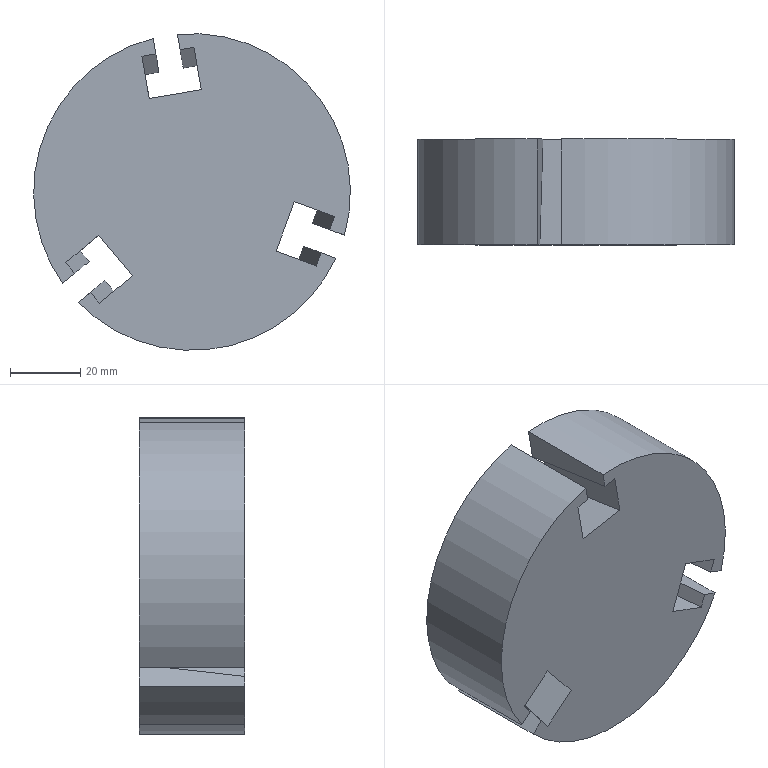Component | SolidWorks | K51-2_K51-3-1 | 1 solid | 27 faces | box 90 x 30 x 90 mm | volume 169880 mm3 | plane 23 | cylinder 4 | commonest cylinder face diameters 90 x4
STEP:
#1=COLOUR_RGB('',0.7922,0.8196,0.9333);
#2=FILL_AREA_STYLE_COLOUR('',#1);
#3=FILL_AREA_STYLE('',(#2));
#4=SURFACE_STYLE_FILL_AREA(#3);
#5=SURFACE_SIDE_STYLE('',(#4));
#6=SURFACE_STYLE_USAGE(.BOTH.,#5);
#7=PRESENTATION_STYLE_ASSIGNMENT((#6));
#8=CARTESIAN_POINT('',(-10.063,38.924,1.881));
#9=VERTEX_POINT('',#8);
#10=CARTESIAN_POINT('',(-10.719,38.924,2.308));
#11=VERTEX_POINT('',#10);
#12=CARTESIAN_POINT('',(-9.449,38.924,3.543));
#13=DIRECTION('',(0.,1.,0.));
#14=DIRECTION('',(0.3464,0.,0.9381));
#15=AXIS2_PLACEMENT_3D('',#12,#13,#14);
#16=CIRCLE('',#15,1.772);
#17=EDGE_CURVE('',#9,#11,#16,.T.);
#18=ORIENTED_EDGE('',*,*,#17,.F.);
#19=CARTESIAN_POINT('',(-10.063,37.743,1.881));
#20=VERTEX_POINT('',#19);
#21=CARTESIAN_POINT('',(-10.063,38.924,1.881));
#22=DIRECTION('',(0.,-1.,0.));
#23=VECTOR('',#22,39.37);
#24=LINE('',#21,#23);
#25=EDGE_CURVE('',#9,#20,#24,.T.);
#26=ORIENTED_EDGE('',*,*,#25,.T.);
#27=CARTESIAN_POINT('',(-10.719,37.743,2.308));
#28=VERTEX_POINT('',#27);
#29=CARTESIAN_POINT('',(-9.449,37.743,3.543));
#30=DIRECTION('',(0.,1.,0.));
#31=DIRECTION('',(0.3464,0.,0.9381));
#32=AXIS2_PLACEMENT_3D('',#29,#30,#31);
#33=CIRCLE('',#32,1.772);
#34=EDGE_CURVE('',#20,#28,#33,.T.);
#35=ORIENTED_EDGE('',*,*,#34,.T.);
#36=CARTESIAN_POINT('',(-10.719,38.924,2.308));
#37=DIRECTION('',(0.,1.,0.));
#38=VECTOR('',#37,39.37);
#39=LINE('',#36,#38);
#40=EDGE_CURVE('',#28,#11,#39,.T.);
#41=ORIENTED_EDGE('',*,*,#40,.T.);
#42=EDGE_LOOP('',(#18,#26,#35,#41));
#43=FACE_OUTER_BOUND('',#42,.T.);
#44=CARTESIAN_POINT('',(-9.449,38.924,3.543));
#45=DIRECTION('',(0.,-1.,0.));
#46=DIRECTION('',(-0.3464,0.,-0.9381));
#47=AXIS2_PLACEMENT_3D('',#44,#45,#46);
#48=CYLINDRICAL_SURFACE('',#47,1.772);
#49=ADVANCED_FACE('',(#43),#48,.T.);
#50=CARTESIAN_POINT('',(-10.895,38.924,2.52));
#51=VERTEX_POINT('',#50);
#52=CARTESIAN_POINT('',(-9.883,38.924,5.261));
#53=VERTEX_POINT('',#52);
#54=CARTESIAN_POINT('',(-9.449,38.924,3.543));
#55=DIRECTION('',(0.,1.,0.));
#56=DIRECTION('',(0.3464,0.,0.9381));
#57=AXIS2_PLACEMENT_3D('',#54,#55,#56);
#58=CIRCLE('',#57,1.772);
#59=EDGE_CURVE('',#51,#53,#58,.T.);
#60=ORIENTED_EDGE('',*,*,#59,.F.);
#61=CARTESIAN_POINT('',(-10.895,37.743,2.52));
#62=VERTEX_POINT('',#61);
#63=CARTESIAN_POINT('',(-10.895,38.924,2.52));
#64=DIRECTION('',(0.,-1.,0.));
#65=VECTOR('',#64,39.37);
#66=LINE('',#63,#65);
#67=EDGE_CURVE('',#51,#62,#66,.T.);
#68=ORIENTED_EDGE('',*,*,#67,.T.);
#69=CARTESIAN_POINT('',(-9.883,37.743,5.261));
#70=VERTEX_POINT('',#69);
#71=CARTESIAN_POINT('',(-9.449,37.743,3.543));
#72=DIRECTION('',(0.,1.,0.));
#73=DIRECTION('',(0.3464,0.,0.9381));
#74=AXIS2_PLACEMENT_3D('',#71,#72,#73);
#75=CIRCLE('',#74,1.772);
#76=EDGE_CURVE('',#62,#70,#75,.T.);
#77=ORIENTED_EDGE('',*,*,#76,.T.);
#78=CARTESIAN_POINT('',(-9.883,38.924,5.261));
#79=DIRECTION('',(0.,1.,0.));
#80=VECTOR('',#79,39.37);
#81=LINE('',#78,#80);
#82=EDGE_CURVE('',#70,#53,#81,.T.);
#83=ORIENTED_EDGE('',*,*,#82,.T.);
#84=EDGE_LOOP('',(#60,#68,#77,#83));
#85=FACE_OUTER_BOUND('',#84,.T.);
#86=CARTESIAN_POINT('',(-9.449,38.924,3.543));
#87=DIRECTION('',(0.,-1.,0.));
#88=DIRECTION('',(-0.3464,0.,-0.9381));
#89=AXIS2_PLACEMENT_3D('',#86,#87,#88);
#90=CYLINDRICAL_SURFACE('',#89,1.772);
#91=ADVANCED_FACE('',(#85),#90,.T.);
#92=CARTESIAN_POINT('',(-9.612,38.924,5.307));
#93=VERTEX_POINT('',#92);
#94=CARTESIAN_POINT('',(-7.744,38.924,3.061));
#95=VERTEX_POINT('',#94);
#96=CARTESIAN_POINT('',(-9.449,38.924,3.543));
#97=DIRECTION('',(0.,1.,0.));
#98=DIRECTION('',(0.3464,0.,0.9381));
#99=AXIS2_PLACEMENT_3D('',#96,#97,#98);
#100=CIRCLE('',#99,1.772);
#101=EDGE_CURVE('',#93,#95,#100,.T.);
#102=ORIENTED_EDGE('',*,*,#101,.F.);
#103=CARTESIAN_POINT('',(-9.612,37.743,5.307));
#104=VERTEX_POINT('',#103);
#105=CARTESIAN_POINT('',(-9.612,38.924,5.307));
#106=DIRECTION('',(0.,-1.,0.));
#107=VECTOR('',#106,39.37);
#108=LINE('',#105,#107);
#109=EDGE_CURVE('',#93,#104,#108,.T.);
#110=ORIENTED_EDGE('',*,*,#109,.T.);
#111=CARTESIAN_POINT('',(-7.744,37.743,3.061));
#112=VERTEX_POINT('',#111);
#113=CARTESIAN_POINT('',(-9.449,37.743,3.543));
#114=DIRECTION('',(0.,1.,0.));
#115=DIRECTION('',(0.3464,0.,0.9381));
#116=AXIS2_PLACEMENT_3D('',#113,#114,#115);
#117=CIRCLE('',#116,1.772);
#118=EDGE_CURVE('',#104,#112,#117,.T.);
#119=ORIENTED_EDGE('',*,*,#118,.T.);
#120=CARTESIAN_POINT('',(-7.744,38.924,3.061));
#121=DIRECTION('',(0.,1.,0.));
#122=VECTOR('',#121,39.37);
#123=LINE('',#120,#122);
#124=EDGE_CURVE('',#112,#95,#123,.T.);
#125=ORIENTED_EDGE('',*,*,#124,.T.);
#126=EDGE_LOOP('',(#102,#110,#119,#125));
#127=FACE_OUTER_BOUND('',#126,.T.);
#128=CARTESIAN_POINT('',(-9.449,38.924,3.543));
#129=DIRECTION('',(0.,-1.,0.));
#130=DIRECTION('',(-0.3464,0.,-0.9381));
#131=AXIS2_PLACEMENT_3D('',#128,#129,#130);
#132=CYLINDRICAL_SURFACE('',#131,1.772);
#133=ADVANCED_FACE('',(#127),#132,.T.);
#134=ORIENTED_EDGE('',*,*,#25,.F.);
#135=CARTESIAN_POINT('',(-7.84,38.924,2.802));
#136=VERTEX_POINT('',#135);
#137=CARTESIAN_POINT('',(-9.449,38.924,3.543));
#138=DIRECTION('',(0.,1.,0.));
#139=DIRECTION('',(0.3464,0.,0.9381));
#140=AXIS2_PLACEMENT_3D('',#137,#138,#139);
#141=CIRCLE('',#140,1.772);
#142=EDGE_CURVE('',#136,#9,#141,.T.);
#143=ORIENTED_EDGE('',*,*,#142,.F.);
#144=CARTESIAN_POINT('',(-7.84,37.743,2.802));
#145=VERTEX_POINT('',#144);
#146=CARTESIAN_POINT('',(-7.84,38.924,2.802));
#147=DIRECTION('',(0.,-1.,0.));
#148=VECTOR('',#147,39.37);
#149=LINE('',#146,#148);
#150=EDGE_CURVE('',#136,#145,#149,.T.);
#151=ORIENTED_EDGE('',*,*,#150,.T.);
#152=CARTESIAN_POINT('',(-9.449,37.743,3.543));
#153=DIRECTION('',(0.,1.,0.));
#154=DIRECTION('',(0.3464,0.,0.9381));
#155=AXIS2_PLACEMENT_3D('',#152,#153,#154);
#156=CIRCLE('',#155,1.772);
#157=EDGE_CURVE('',#145,#20,#156,.T.);
#158=ORIENTED_EDGE('',*,*,#157,.T.);
#159=EDGE_LOOP('',(#134,#143,#151,#158));
#160=FACE_OUTER_BOUND('',#159,.T.);
#161=CARTESIAN_POINT('',(-9.449,38.924,3.543));
#162=DIRECTION('',(0.,-1.,0.));
#163=DIRECTION('',(-0.3464,0.,-0.9381));
#164=AXIS2_PLACEMENT_3D('',#161,#162,#163);
#165=CYLINDRICAL_SURFACE('',#164,1.772);
#166=ADVANCED_FACE('',(#160),#165,.T.);
#167=CARTESIAN_POINT('',(-10.601,38.924,2.765));
#168=VERTEX_POINT('',#167);
#169=CARTESIAN_POINT('',(-9.537,38.924,3.649));
#170=DIRECTION('',(0.769,0.,0.6392));
#171=VECTOR('',#170,39.37);
#172=LINE('',#169,#171);
#173=EDGE_CURVE('',#51,#168,#172,.T.);
#174=ORIENTED_EDGE('',*,*,#173,.F.);
#175=ORIENTED_EDGE('',*,*,#59,.T.);
#176=CARTESIAN_POINT('',(-9.818,38.924,4.883));
#177=VERTEX_POINT('',#176);
#178=CARTESIAN_POINT('',(-9.585,38.924,3.52));
#179=DIRECTION('',(-0.169,0.,0.9856));
#180=VECTOR('',#179,39.37);
#181=LINE('',#178,#180);
#182=EDGE_CURVE('',#177,#53,#181,.T.);
#183=ORIENTED_EDGE('',*,*,#182,.F.);
#184=CARTESIAN_POINT('',(-9.974,38.924,4.857));
#185=VERTEX_POINT('',#184);
#186=CARTESIAN_POINT('',(-9.683,38.924,4.907));
#187=DIRECTION('',(0.9856,0.,0.169));
#188=VECTOR('',#187,39.37);
#189=LINE('',#186,#188);
#190=EDGE_CURVE('',#185,#177,#189,.T.);
#191=ORIENTED_EDGE('',*,*,#190,.F.);
#192=CARTESIAN_POINT('',(-9.893,38.924,4.384));
#193=VERTEX_POINT('',#192);
#194=CARTESIAN_POINT('',(-9.74,38.924,3.493));
#195=DIRECTION('',(-0.169,0.,0.9856));
#196=VECTOR('',#195,39.37);
#197=LINE('',#194,#196);
#198=EDGE_CURVE('',#193,#185,#197,.T.);
#199=ORIENTED_EDGE('',*,*,#198,.F.);
#200=CARTESIAN_POINT('',(-9.31,38.924,4.484));
#201=VERTEX_POINT('',#200);
#202=CARTESIAN_POINT('',(-9.602,38.924,4.434));
#203=DIRECTION('',(-0.9856,0.,-0.169));
#204=VECTOR('',#203,39.37);
#205=LINE('',#202,#204);
#206=EDGE_CURVE('',#201,#193,#205,.T.);
#207=ORIENTED_EDGE('',*,*,#206,.F.);
#208=CARTESIAN_POINT('',(-9.392,38.924,4.956));
#209=VERTEX_POINT('',#208);
#210=CARTESIAN_POINT('',(-9.158,38.924,3.593));
#211=DIRECTION('',(0.169,0.,-0.9856));
#212=VECTOR('',#211,39.37);
#213=LINE('',#210,#212);
#214=EDGE_CURVE('',#209,#201,#213,.T.);
#215=ORIENTED_EDGE('',*,*,#214,.F.);
#216=CARTESIAN_POINT('',(-9.547,38.924,4.93));
#217=VERTEX_POINT('',#216);
#218=CARTESIAN_POINT('',(-9.683,38.924,4.907));
#219=DIRECTION('',(0.9856,0.,0.169));
#220=VECTOR('',#219,39.37);
#221=LINE('',#218,#220);
#222=EDGE_CURVE('',#217,#209,#221,.T.);
#223=ORIENTED_EDGE('',*,*,#222,.F.);
#224=CARTESIAN_POINT('',(-9.313,38.924,3.567));
#225=DIRECTION('',(0.169,0.,-0.9856));
#226=VECTOR('',#225,39.37);
#227=LINE('',#224,#226);
#228=EDGE_CURVE('',#93,#217,#227,.T.);
#229=ORIENTED_EDGE('',*,*,#228,.F.);
#230=ORIENTED_EDGE('',*,*,#101,.T.);
#231=CARTESIAN_POINT('',(-8.104,38.924,3.193));
#232=VERTEX_POINT('',#231);
#233=CARTESIAN_POINT('',(-9.401,38.924,3.673));
#234=DIRECTION('',(0.9381,0.,-0.3464));
#235=VECTOR('',#234,39.37);
#236=LINE('',#233,#235);
#237=EDGE_CURVE('',#232,#95,#236,.T.);
#238=ORIENTED_EDGE('',*,*,#237,.F.);
#239=CARTESIAN_POINT('',(-8.049,38.924,3.341));
#240=VERTEX_POINT('',#239);
#241=CARTESIAN_POINT('',(-8.151,38.924,3.064));
#242=DIRECTION('',(-0.3464,0.,-0.9381));
#243=VECTOR('',#242,39.37);
#244=LINE('',#241,#243);
#245=EDGE_CURVE('',#240,#232,#244,.T.);
#246=ORIENTED_EDGE('',*,*,#245,.F.);
#247=CARTESIAN_POINT('',(-8.499,38.924,3.507));
#248=VERTEX_POINT('',#247);
#249=CARTESIAN_POINT('',(-9.347,38.924,3.82));
#250=DIRECTION('',(0.9381,0.,-0.3464));
#251=VECTOR('',#250,39.37);
#252=LINE('',#249,#251);
#253=EDGE_CURVE('',#248,#240,#252,.T.);
#254=ORIENTED_EDGE('',*,*,#253,.F.);
#255=CARTESIAN_POINT('',(-8.704,38.924,2.953));
#256=VERTEX_POINT('',#255);
#257=CARTESIAN_POINT('',(-8.601,38.924,3.23));
#258=DIRECTION('',(0.3464,0.,0.9381));
#259=VECTOR('',#258,39.37);
#260=LINE('',#257,#259);
#261=EDGE_CURVE('',#256,#248,#260,.T.);
#262=ORIENTED_EDGE('',*,*,#261,.F.);
#263=CARTESIAN_POINT('',(-8.254,38.924,2.787));
#264=VERTEX_POINT('',#263);
#265=CARTESIAN_POINT('',(-9.551,38.924,3.266));
#266=DIRECTION('',(-0.9381,0.,0.3464));
#267=VECTOR('',#266,39.37);
#268=LINE('',#265,#267);
#269=EDGE_CURVE('',#264,#256,#268,.T.);
#270=ORIENTED_EDGE('',*,*,#269,.F.);
#271=CARTESIAN_POINT('',(-8.199,38.924,2.935));
#272=VERTEX_POINT('',#271);
#273=CARTESIAN_POINT('',(-8.151,38.924,3.064));
#274=DIRECTION('',(-0.3464,0.,-0.9381));
#275=VECTOR('',#274,39.37);
#276=LINE('',#273,#275);
#277=EDGE_CURVE('',#272,#264,#276,.T.);
#278=ORIENTED_EDGE('',*,*,#277,.F.);
#279=CARTESIAN_POINT('',(-9.497,38.924,3.414));
#280=DIRECTION('',(-0.9381,0.,0.3464));
#281=VECTOR('',#280,39.37);
#282=LINE('',#279,#281);
#283=EDGE_CURVE('',#136,#272,#282,.T.);
#284=ORIENTED_EDGE('',*,*,#283,.F.);
#285=ORIENTED_EDGE('',*,*,#142,.T.);
#286=ORIENTED_EDGE('',*,*,#17,.T.);
#287=CARTESIAN_POINT('',(-10.424,38.924,2.553));
#288=VERTEX_POINT('',#287);
#289=CARTESIAN_POINT('',(-9.361,38.924,3.437));
#290=DIRECTION('',(-0.769,0.,-0.6392));
#291=VECTOR('',#290,39.37);
#292=LINE('',#289,#291);
#293=EDGE_CURVE('',#288,#11,#292,.T.);
#294=ORIENTED_EDGE('',*,*,#293,.F.);
#295=CARTESIAN_POINT('',(-10.324,38.924,2.432));
#296=VERTEX_POINT('',#295);
#297=CARTESIAN_POINT('',(-10.513,38.924,2.659));
#298=DIRECTION('',(-0.6392,0.,0.769));
#299=VECTOR('',#298,39.37);
#300=LINE('',#297,#299);
#301=EDGE_CURVE('',#296,#288,#300,.T.);
#302=ORIENTED_EDGE('',*,*,#301,.F.);
#303=CARTESIAN_POINT('',(-9.955,38.924,2.739));
#304=VERTEX_POINT('',#303);
#305=CARTESIAN_POINT('',(-9.26,38.924,3.316));
#306=DIRECTION('',(-0.769,0.,-0.6392));
#307=VECTOR('',#306,39.37);
#308=LINE('',#305,#307);
#309=EDGE_CURVE('',#304,#296,#308,.T.);
#310=ORIENTED_EDGE('',*,*,#309,.F.);
#311=CARTESIAN_POINT('',(-10.332,38.924,3.193));
#312=VERTEX_POINT('',#311);
#313=CARTESIAN_POINT('',(-10.144,38.924,2.966));
#314=DIRECTION('',(0.6392,0.,-0.769));
#315=VECTOR('',#314,39.37);
#316=LINE('',#313,#315);
#317=EDGE_CURVE('',#312,#304,#316,.T.);
#318=ORIENTED_EDGE('',*,*,#317,.F.);
#319=CARTESIAN_POINT('',(-10.701,38.924,2.886));
#320=VERTEX_POINT('',#319);
#321=CARTESIAN_POINT('',(-9.638,38.924,3.77));
#322=DIRECTION('',(0.769,0.,0.6392));
#323=VECTOR('',#322,39.37);
#324=LINE('',#321,#323);
#325=EDGE_CURVE('',#320,#312,#324,.T.);
#326=ORIENTED_EDGE('',*,*,#325,.F.);
#327=CARTESIAN_POINT('',(-10.513,38.924,2.659));
#328=DIRECTION('',(-0.6392,0.,0.769));
#329=VECTOR('',#328,39.37);
#330=LINE('',#327,#329);
#331=EDGE_CURVE('',#168,#320,#330,.T.);
#332=ORIENTED_EDGE('',*,*,#331,.F.);
#333=EDGE_LOOP('',(#174,#175,#183,#191,#199,#207,#215,#223,#229,#230,#238,#246,#254,#262,#270,#278,#284,#285,#286,#294,#302,#310,#318,#326,#332));
#334=FACE_OUTER_BOUND('',#333,.T.);
#335=CARTESIAN_POINT('',(-9.449,38.924,3.543));
#336=DIRECTION('',(0.,1.,0.));
#337=DIRECTION('',(0.3464,0.,0.9381));
#338=AXIS2_PLACEMENT_3D('',#335,#336,#337);
#339=PLANE('',#338);
#340=ADVANCED_FACE('',(#334),#339,.T.);
#341=ORIENTED_EDGE('',*,*,#76,.F.);
#342=CARTESIAN_POINT('',(-10.761,37.743,2.632));
#343=VERTEX_POINT('',#342);
#344=CARTESIAN_POINT('',(-9.537,37.743,3.649));
#345=DIRECTION('',(0.769,0.,0.6392));
#346=VECTOR('',#345,39.37);
#347=LINE('',#344,#346);
#348=EDGE_CURVE('',#62,#343,#347,.T.);
#349=ORIENTED_EDGE('',*,*,#348,.T.);
#350=CARTESIAN_POINT('',(-10.861,37.743,2.753));
#351=VERTEX_POINT('',#350);
#352=CARTESIAN_POINT('',(-10.673,37.743,2.526));
#353=DIRECTION('',(-0.6392,0.,0.769));
#354=VECTOR('',#353,39.37);
#355=LINE('',#352,#354);
#356=EDGE_CURVE('',#343,#351,#355,.T.);
#357=ORIENTED_EDGE('',*,*,#356,.T.);
#358=CARTESIAN_POINT('',(-10.492,37.743,3.06));
#359=VERTEX_POINT('',#358);
#360=CARTESIAN_POINT('',(-9.638,37.743,3.77));
#361=DIRECTION('',(0.769,0.,0.6392));
#362=VECTOR('',#361,39.37);
#363=LINE('',#360,#362);
#364=EDGE_CURVE('',#351,#359,#363,.T.);
#365=ORIENTED_EDGE('',*,*,#364,.T.);
#366=CARTESIAN_POINT('',(-10.115,37.743,2.606));
#367=VERTEX_POINT('',#366);
#368=CARTESIAN_POINT('',(-10.304,37.743,2.833));
#369=DIRECTION('',(0.6392,0.,-0.769));
#370=VECTOR('',#369,39.37);
#371=LINE('',#368,#370);
#372=EDGE_CURVE('',#359,#367,#371,.T.);
#373=ORIENTED_EDGE('',*,*,#372,.T.);
#374=CARTESIAN_POINT('',(-10.484,37.743,2.299));
#375=VERTEX_POINT('',#374);
#376=CARTESIAN_POINT('',(-9.26,37.743,3.316));
#377=DIRECTION('',(-0.769,0.,-0.6392));
#378=VECTOR('',#377,39.37);
#379=LINE('',#376,#378);
#380=EDGE_CURVE('',#367,#375,#379,.T.);
#381=ORIENTED_EDGE('',*,*,#380,.T.);
#382=CARTESIAN_POINT('',(-10.585,37.743,2.42));
#383=VERTEX_POINT('',#382);
#384=CARTESIAN_POINT('',(-10.673,37.743,2.526));
#385=DIRECTION('',(-0.6392,0.,0.769));
#386=VECTOR('',#385,39.37);
#387=LINE('',#384,#386);
#388=EDGE_CURVE('',#375,#383,#387,.T.);
#389=ORIENTED_EDGE('',*,*,#388,.T.);
#390=CARTESIAN_POINT('',(-9.361,37.743,3.437));
#391=DIRECTION('',(-0.769,0.,-0.6392));
#392=VECTOR('',#391,39.37);
#393=LINE('',#390,#392);
#394=EDGE_CURVE('',#383,#28,#393,.T.);
#395=ORIENTED_EDGE('',*,*,#394,.T.);
#396=ORIENTED_EDGE('',*,*,#34,.F.);
#397=ORIENTED_EDGE('',*,*,#157,.F.);
#398=CARTESIAN_POINT('',(-8.004,37.743,2.863));
#399=VERTEX_POINT('',#398);
#400=CARTESIAN_POINT('',(-9.497,37.743,3.414));
#401=DIRECTION('',(-0.9381,0.,0.3464));
#402=VECTOR('',#401,39.37);
#403=LINE('',#400,#402);
#404=EDGE_CURVE('',#145,#399,#403,.T.);
#405=ORIENTED_EDGE('',*,*,#404,.T.);
#406=CARTESIAN_POINT('',(-8.058,37.743,2.715));
#407=VERTEX_POINT('',#406);
#408=CARTESIAN_POINT('',(-7.956,37.743,2.992));
#409=DIRECTION('',(-0.3464,0.,-0.9381));
#410=VECTOR('',#409,39.37);
#411=LINE('',#408,#410);
#412=EDGE_CURVE('',#399,#407,#411,.T.);
#413=ORIENTED_EDGE('',*,*,#412,.T.);
#414=CARTESIAN_POINT('',(-8.508,37.743,2.881));
#415=VERTEX_POINT('',#414);
#416=CARTESIAN_POINT('',(-9.551,37.743,3.266));
#417=DIRECTION('',(-0.9381,0.,0.3464));
#418=VECTOR('',#417,39.37);
#419=LINE('',#416,#418);
#420=EDGE_CURVE('',#407,#415,#419,.T.);
#421=ORIENTED_EDGE('',*,*,#420,.T.);
#422=CARTESIAN_POINT('',(-8.304,37.743,3.435));
#423=VERTEX_POINT('',#422);
#424=CARTESIAN_POINT('',(-8.406,37.743,3.158));
#425=DIRECTION('',(0.3464,0.,0.9381));
#426=VECTOR('',#425,39.37);
#427=LINE('',#424,#426);
#428=EDGE_CURVE('',#415,#423,#427,.T.);
#429=ORIENTED_EDGE('',*,*,#428,.T.);
#430=CARTESIAN_POINT('',(-7.854,37.743,3.269));
#431=VERTEX_POINT('',#430);
#432=CARTESIAN_POINT('',(-9.347,37.743,3.82));
#433=DIRECTION('',(0.9381,0.,-0.3464));
#434=VECTOR('',#433,39.37);
#435=LINE('',#432,#434);
#436=EDGE_CURVE('',#423,#431,#435,.T.);
#437=ORIENTED_EDGE('',*,*,#436,.T.);
#438=CARTESIAN_POINT('',(-7.908,37.743,3.121));
#439=VERTEX_POINT('',#438);
#440=CARTESIAN_POINT('',(-7.956,37.743,2.992));
#441=DIRECTION('',(-0.3464,0.,-0.9381));
#442=VECTOR('',#441,39.37);
#443=LINE('',#440,#442);
#444=EDGE_CURVE('',#431,#439,#443,.T.);
#445=ORIENTED_EDGE('',*,*,#444,.T.);
#446=CARTESIAN_POINT('',(-9.401,37.743,3.673));
#447=DIRECTION('',(0.9381,0.,-0.3464));
#448=VECTOR('',#447,39.37);
#449=LINE('',#446,#448);
#450=EDGE_CURVE('',#439,#112,#449,.T.);
#451=ORIENTED_EDGE('',*,*,#450,.T.);
#452=ORIENTED_EDGE('',*,*,#118,.F.);
#453=CARTESIAN_POINT('',(-9.582,37.743,5.135));
#454=VERTEX_POINT('',#453);
#455=CARTESIAN_POINT('',(-9.313,37.743,3.567));
#456=DIRECTION('',(0.169,0.,-0.9856));
#457=VECTOR('',#456,39.37);
#458=LINE('',#455,#457);
#459=EDGE_CURVE('',#104,#454,#458,.T.);
#460=ORIENTED_EDGE('',*,*,#459,.T.);
#461=CARTESIAN_POINT('',(-9.427,37.743,5.162));
#462=VERTEX_POINT('',#461);
#463=CARTESIAN_POINT('',(-9.718,37.743,5.112));
#464=DIRECTION('',(0.9856,0.,0.169));
#465=VECTOR('',#464,39.37);
#466=LINE('',#463,#465);
#467=EDGE_CURVE('',#454,#462,#466,.T.);
#468=ORIENTED_EDGE('',*,*,#467,.T.);
#469=CARTESIAN_POINT('',(-9.346,37.743,4.689));
#470=VERTEX_POINT('',#469);
#471=CARTESIAN_POINT('',(-9.158,37.743,3.593));
#472=DIRECTION('',(0.169,0.,-0.9856));
#473=VECTOR('',#472,39.37);
#474=LINE('',#471,#473);
#475=EDGE_CURVE('',#462,#470,#474,.T.);
#476=ORIENTED_EDGE('',*,*,#475,.T.);
#477=CARTESIAN_POINT('',(-9.928,37.743,4.589));
#478=VERTEX_POINT('',#477);
#479=CARTESIAN_POINT('',(-9.637,37.743,4.639));
#480=DIRECTION('',(-0.9856,0.,-0.169));
#481=VECTOR('',#480,39.37);
#482=LINE('',#479,#481);
#483=EDGE_CURVE('',#470,#478,#482,.T.);
#484=ORIENTED_EDGE('',*,*,#483,.T.);
#485=CARTESIAN_POINT('',(-10.009,37.743,5.062));
#486=VERTEX_POINT('',#485);
#487=CARTESIAN_POINT('',(-9.74,37.743,3.493));
#488=DIRECTION('',(-0.169,0.,0.9856));
#489=VECTOR('',#488,39.37);
#490=LINE('',#487,#489);
#491=EDGE_CURVE('',#478,#486,#490,.T.);
#492=ORIENTED_EDGE('',*,*,#491,.T.);
#493=CARTESIAN_POINT('',(-9.854,37.743,5.089));
#494=VERTEX_POINT('',#493);
#495=CARTESIAN_POINT('',(-9.718,37.743,5.112));
#496=DIRECTION('',(0.9856,0.,0.169));
#497=VECTOR('',#496,39.37);
#498=LINE('',#495,#497);
#499=EDGE_CURVE('',#486,#494,#498,.T.);
#500=ORIENTED_EDGE('',*,*,#499,.T.);
#501=CARTESIAN_POINT('',(-9.585,37.743,3.52));
#502=DIRECTION('',(-0.169,0.,0.9856));
#503=VECTOR('',#502,39.37);
#504=LINE('',#501,#503);
#505=EDGE_CURVE('',#494,#70,#504,.T.);
#506=ORIENTED_EDGE('',*,*,#505,.T.);
#507=EDGE_LOOP('',(#341,#349,#357,#365,#373,#381,#389,#395,#396,#397,#405,#413,#421,#429,#437,#445,#451,#452,#460,#468,#476,#484,#492,#500,#506));
#508=FACE_OUTER_BOUND('',#507,.T.);
#509=CARTESIAN_POINT('',(-9.449,37.743,3.543));
#510=DIRECTION('',(0.,1.,0.));
#511=DIRECTION('',(0.3464,0.,0.9381));
#512=AXIS2_PLACEMENT_3D('',#509,#510,#511);
#513=PLANE('',#512);
#514=ADVANCED_FACE('',(#508),#513,.F.);
#515=ORIENTED_EDGE('',*,*,#269,.T.);
#516=CARTESIAN_POINT('',(-8.225,36.03,2.777));
#517=DIRECTION('',(-0.1629,0.9848,0.06016));
#518=VECTOR('',#517,39.37);
#519=LINE('',#516,#518);
#520=EDGE_CURVE('',#415,#256,#519,.T.);
#521=ORIENTED_EDGE('',*,*,#520,.F.);
#522=ORIENTED_EDGE('',*,*,#420,.F.);
#523=CARTESIAN_POINT('',(-7.789,36.112,2.615));
#524=DIRECTION('',(-0.1629,0.9848,0.06016));
#525=VECTOR('',#524,39.37);
#526=LINE('',#523,#525);
#527=EDGE_CURVE('',#407,#264,#526,.T.);
#528=ORIENTED_EDGE('',*,*,#527,.T.);
#529=EDGE_LOOP('',(#515,#521,#522,#528));
#530=FACE_OUTER_BOUND('',#529,.T.);
#531=CARTESIAN_POINT('',(-7.789,36.112,2.615));
#532=DIRECTION('',(-0.3464,-0.,-0.9381));
#533=DIRECTION('',(-0.9381,0.,0.3464));
#534=AXIS2_PLACEMENT_3D('',#531,#532,#533);
#535=PLANE('',#534);
#536=ADVANCED_FACE('',(#530),#535,.F.);
#537=ORIENTED_EDGE('',*,*,#277,.T.);
#538=ORIENTED_EDGE('',*,*,#527,.F.);
#539=ORIENTED_EDGE('',*,*,#412,.F.);
#540=CARTESIAN_POINT('',(-7.734,36.112,2.763));
#541=DIRECTION('',(-0.1629,0.9848,0.06016));
#542=VECTOR('',#541,39.37);
#543=LINE('',#540,#542);
#544=EDGE_CURVE('',#399,#272,#543,.T.);
#545=ORIENTED_EDGE('',*,*,#544,.T.);
#546=EDGE_LOOP('',(#537,#538,#539,#545));
#547=FACE_OUTER_BOUND('',#546,.T.);
#548=CARTESIAN_POINT('',(-7.734,36.112,2.763));
#549=DIRECTION('',(0.9238,0.1736,-0.3412));
#550=DIRECTION('',(-0.1629,0.9848,0.06016));
#551=AXIS2_PLACEMENT_3D('',#548,#549,#550);
#552=PLANE('',#551);
#553=ADVANCED_FACE('',(#547),#552,.F.);
#554=ORIENTED_EDGE('',*,*,#245,.T.);
#555=CARTESIAN_POINT('',(-7.639,36.112,3.022));
#556=DIRECTION('',(-0.1629,0.9848,0.06016));
#557=VECTOR('',#556,39.37);
#558=LINE('',#555,#557);
#559=EDGE_CURVE('',#439,#232,#558,.T.);
#560=ORIENTED_EDGE('',*,*,#559,.F.);
#561=ORIENTED_EDGE('',*,*,#444,.F.);
#562=CARTESIAN_POINT('',(-7.584,36.112,3.169));
#563=DIRECTION('',(-0.1629,0.9848,0.06016));
#564=VECTOR('',#563,39.37);
#565=LINE('',#562,#564);
#566=EDGE_CURVE('',#431,#240,#565,.T.);
#567=ORIENTED_EDGE('',*,*,#566,.T.);
#568=EDGE_LOOP('',(#554,#560,#561,#567));
#569=FACE_OUTER_BOUND('',#568,.T.);
#570=CARTESIAN_POINT('',(-7.584,36.112,3.169));
#571=DIRECTION('',(0.9238,0.1736,-0.3412));
#572=DIRECTION('',(-0.1629,0.9848,0.06016));
#573=AXIS2_PLACEMENT_3D('',#570,#571,#572);
#574=PLANE('',#573);
#575=ADVANCED_FACE('',(#569),#574,.F.);
#576=ORIENTED_EDGE('',*,*,#253,.T.);
#577=ORIENTED_EDGE('',*,*,#566,.F.);
#578=ORIENTED_EDGE('',*,*,#436,.F.);
#579=CARTESIAN_POINT('',(-8.02,36.03,3.331));
#580=DIRECTION('',(-0.1629,0.9848,0.06016));
#581=VECTOR('',#580,39.37);
#582=LINE('',#579,#581);
#583=EDGE_CURVE('',#423,#248,#582,.T.);
#584=ORIENTED_EDGE('',*,*,#583,.T.);
#585=EDGE_LOOP('',(#576,#577,#578,#584));
#586=FACE_OUTER_BOUND('',#585,.T.);
#587=CARTESIAN_POINT('',(-8.02,36.03,3.331));
#588=DIRECTION('',(0.3464,0.,0.9381));
#589=DIRECTION('',(0.9381,0.,-0.3464));
#590=AXIS2_PLACEMENT_3D('',#587,#588,#589);
#591=PLANE('',#590);
#592=ADVANCED_FACE('',(#586),#591,.F.);
#593=ORIENTED_EDGE('',*,*,#261,.T.);
#594=ORIENTED_EDGE('',*,*,#583,.F.);
#595=ORIENTED_EDGE('',*,*,#428,.F.);
#596=ORIENTED_EDGE('',*,*,#520,.T.);
#597=EDGE_LOOP('',(#593,#594,#595,#596));
#598=FACE_OUTER_BOUND('',#597,.T.);
#599=CARTESIAN_POINT('',(-8.225,36.03,2.777));
#600=DIRECTION('',(-0.9238,-0.1736,0.3412));
#601=DIRECTION('',(0.1629,-0.9848,-0.06016));
#602=AXIS2_PLACEMENT_3D('',#599,#600,#601);
#603=PLANE('',#602);
#604=ADVANCED_FACE('',(#598),#603,.F.);
#605=ORIENTED_EDGE('',*,*,#283,.T.);
#606=ORIENTED_EDGE('',*,*,#544,.F.);
#607=ORIENTED_EDGE('',*,*,#404,.F.);
#608=ORIENTED_EDGE('',*,*,#150,.F.);
#609=EDGE_LOOP('',(#605,#606,#607,#608));
#610=FACE_OUTER_BOUND('',#609,.T.);
#611=CARTESIAN_POINT('',(-7.083,36.235,2.523));
#612=DIRECTION('',(-0.3464,-0.,-0.9381));
#613=DIRECTION('',(-0.9381,0.,0.3464));
#614=AXIS2_PLACEMENT_3D('',#611,#612,#613);
#615=PLANE('',#614);
#616=ADVANCED_FACE('',(#610),#615,.F.);
#617=ORIENTED_EDGE('',*,*,#237,.T.);
#618=ORIENTED_EDGE('',*,*,#124,.F.);
#619=ORIENTED_EDGE('',*,*,#450,.F.);
#620=ORIENTED_EDGE('',*,*,#559,.T.);
#621=EDGE_LOOP('',(#617,#618,#619,#620));
#622=FACE_OUTER_BOUND('',#621,.T.);
#623=CARTESIAN_POINT('',(-7.639,36.112,3.022));
#624=DIRECTION('',(0.3464,0.,0.9381));
#625=DIRECTION('',(0.9381,0.,-0.3464));
#626=AXIS2_PLACEMENT_3D('',#623,#624,#625);
#627=PLANE('',#626);
#628=ADVANCED_FACE('',(#622),#627,.F.);
#629=ORIENTED_EDGE('',*,*,#214,.T.);
#630=CARTESIAN_POINT('',(-9.397,36.03,4.987));
#631=DIRECTION('',(0.02935,0.9848,-0.1711));
#632=VECTOR('',#631,39.37);
#633=LINE('',#630,#632);
#634=EDGE_CURVE('',#470,#201,#633,.T.);
#635=ORIENTED_EDGE('',*,*,#634,.F.);
#636=ORIENTED_EDGE('',*,*,#475,.F.);
#637=CARTESIAN_POINT('',(-9.475,36.112,5.445));
#638=DIRECTION('',(0.02935,0.9848,-0.1711));
#639=VECTOR('',#638,39.37);
#640=LINE('',#637,#639);
#641=EDGE_CURVE('',#462,#209,#640,.T.);
#642=ORIENTED_EDGE('',*,*,#641,.T.);
#643=EDGE_LOOP('',(#629,#635,#636,#642));
#644=FACE_OUTER_BOUND('',#643,.T.);
#645=CARTESIAN_POINT('',(-9.475,36.112,5.445));
#646=DIRECTION('',(0.9856,0.,0.169));
#647=DIRECTION('',(0.169,0.,-0.9856));
#648=AXIS2_PLACEMENT_3D('',#645,#646,#647);
#649=PLANE('',#648);
#650=ADVANCED_FACE('',(#644),#649,.F.);
#651=ORIENTED_EDGE('',*,*,#222,.T.);
#652=ORIENTED_EDGE('',*,*,#641,.F.);
#653=ORIENTED_EDGE('',*,*,#467,.F.);
#654=CARTESIAN_POINT('',(-9.631,36.112,5.418));
#655=DIRECTION('',(0.02935,0.9848,-0.1711));
#656=VECTOR('',#655,39.37);
#657=LINE('',#654,#656);
#658=EDGE_CURVE('',#454,#217,#657,.T.);
#659=ORIENTED_EDGE('',*,*,#658,.T.);
#660=EDGE_LOOP('',(#651,#652,#653,#659));
#661=FACE_OUTER_BOUND('',#660,.T.);
#662=CARTESIAN_POINT('',(-9.631,36.112,5.418));
#663=DIRECTION('',(-0.1665,0.1736,0.9706));
#664=DIRECTION('',(0.9856,0.,0.169));
#665=AXIS2_PLACEMENT_3D('',#662,#663,#664);
#666=PLANE('',#665);
#667=ADVANCED_FACE('',(#661),#666,.F.);
#668=ORIENTED_EDGE('',*,*,#190,.T.);
#669=CARTESIAN_POINT('',(-9.902,36.112,5.372));
#670=DIRECTION('',(0.02935,0.9848,-0.1711));
#671=VECTOR('',#670,39.37);
#672=LINE('',#669,#671);
#673=EDGE_CURVE('',#494,#177,#672,.T.);
#674=ORIENTED_EDGE('',*,*,#673,.F.);
#675=ORIENTED_EDGE('',*,*,#499,.F.);
#676=CARTESIAN_POINT('',(-10.057,36.112,5.345));
#677=DIRECTION('',(0.02935,0.9848,-0.1711));
#678=VECTOR('',#677,39.37);
#679=LINE('',#676,#678);
#680=EDGE_CURVE('',#486,#185,#679,.T.);
#681=ORIENTED_EDGE('',*,*,#680,.T.);
#682=EDGE_LOOP('',(#668,#674,#675,#681));
#683=FACE_OUTER_BOUND('',#682,.T.);
#684=CARTESIAN_POINT('',(-10.057,36.112,5.345));
#685=DIRECTION('',(-0.1665,0.1736,0.9706));
#686=DIRECTION('',(0.9856,0.,0.169));
#687=AXIS2_PLACEMENT_3D('',#684,#685,#686);
#688=PLANE('',#687);
#689=ADVANCED_FACE('',(#683),#688,.F.);
#690=ORIENTED_EDGE('',*,*,#198,.T.);
#691=ORIENTED_EDGE('',*,*,#680,.F.);
#692=ORIENTED_EDGE('',*,*,#491,.F.);
#693=CARTESIAN_POINT('',(-9.979,36.03,4.887));
#694=DIRECTION('',(0.02935,0.9848,-0.1711));
#695=VECTOR('',#694,39.37);
#696=LINE('',#693,#695);
#697=EDGE_CURVE('',#478,#193,#696,.T.);
#698=ORIENTED_EDGE('',*,*,#697,.T.);
#699=EDGE_LOOP('',(#690,#691,#692,#698));
#700=FACE_OUTER_BOUND('',#699,.T.);
#701=CARTESIAN_POINT('',(-9.979,36.03,4.887));
#702=DIRECTION('',(-0.9856,-0.,-0.169));
#703=DIRECTION('',(-0.169,0.,0.9856));
#704=AXIS2_PLACEMENT_3D('',#701,#702,#703);
#705=PLANE('',#704);
#706=ADVANCED_FACE('',(#700),#705,.F.);
#707=ORIENTED_EDGE('',*,*,#206,.T.);
#708=ORIENTED_EDGE('',*,*,#697,.F.);
#709=ORIENTED_EDGE('',*,*,#483,.F.);
#710=ORIENTED_EDGE('',*,*,#634,.T.);
#711=EDGE_LOOP('',(#707,#708,#709,#710));
#712=FACE_OUTER_BOUND('',#711,.T.);
#713=CARTESIAN_POINT('',(-9.397,36.03,4.987));
#714=DIRECTION('',(0.1665,-0.1736,-0.9706));
#715=DIRECTION('',(-0.9856,0.,-0.169));
#716=AXIS2_PLACEMENT_3D('',#713,#714,#715);
#717=PLANE('',#716);
#718=ADVANCED_FACE('',(#712),#717,.F.);
#719=ORIENTED_EDGE('',*,*,#228,.T.);
#720=ORIENTED_EDGE('',*,*,#658,.F.);
#721=ORIENTED_EDGE('',*,*,#459,.F.);
#722=ORIENTED_EDGE('',*,*,#109,.F.);
#723=EDGE_LOOP('',(#719,#720,#721,#722));
#724=FACE_OUTER_BOUND('',#723,.T.);
#725=CARTESIAN_POINT('',(-9.748,36.235,6.102));
#726=DIRECTION('',(0.9856,-0.,0.169));
#727=DIRECTION('',(0.169,0.,-0.9856));
#728=AXIS2_PLACEMENT_3D('',#725,#726,#727);
#729=PLANE('',#728);
#730=ADVANCED_FACE('',(#724),#729,.F.);
#731=ORIENTED_EDGE('',*,*,#182,.T.);
#732=ORIENTED_EDGE('',*,*,#82,.F.);
#733=ORIENTED_EDGE('',*,*,#505,.F.);
#734=ORIENTED_EDGE('',*,*,#673,.T.);
#735=EDGE_LOOP('',(#731,#732,#733,#734));
#736=FACE_OUTER_BOUND('',#735,.T.);
#737=CARTESIAN_POINT('',(-9.902,36.112,5.372));
#738=DIRECTION('',(-0.9856,-0.,-0.169));
#739=DIRECTION('',(-0.169,0.,0.9856));
#740=AXIS2_PLACEMENT_3D('',#737,#738,#739);
#741=PLANE('',#740);
#742=ADVANCED_FACE('',(#736),#741,.F.);
#743=ORIENTED_EDGE('',*,*,#325,.T.);
#744=CARTESIAN_POINT('',(-10.725,36.03,2.867));
#745=DIRECTION('',(0.1335,0.9848,0.111));
#746=VECTOR('',#745,39.37);
#747=LINE('',#744,#746);
#748=EDGE_CURVE('',#359,#312,#747,.T.);
#749=ORIENTED_EDGE('',*,*,#748,.F.);
#750=ORIENTED_EDGE('',*,*,#364,.F.);
#751=CARTESIAN_POINT('',(-11.083,36.112,2.569));
#752=DIRECTION('',(0.1335,0.9848,0.111));
#753=VECTOR('',#752,39.37);
#754=LINE('',#751,#753);
#755=EDGE_CURVE('',#351,#320,#754,.T.);
#756=ORIENTED_EDGE('',*,*,#755,.T.);
#757=EDGE_LOOP('',(#743,#749,#750,#756));
#758=FACE_OUTER_BOUND('',#757,.T.);
#759=CARTESIAN_POINT('',(-11.083,36.112,2.569));
#760=DIRECTION('',(-0.6392,-0.,0.769));
#761=DIRECTION('',(0.769,0.,0.6392));
#762=AXIS2_PLACEMENT_3D('',#759,#760,#761);
#763=PLANE('',#762);
#764=ADVANCED_FACE('',(#758),#763,.F.);
#765=ORIENTED_EDGE('',*,*,#331,.T.);
#766=ORIENTED_EDGE('',*,*,#755,.F.);
#767=ORIENTED_EDGE('',*,*,#356,.F.);
#768=CARTESIAN_POINT('',(-10.982,36.112,2.448));
#769=DIRECTION('',(0.1335,0.9848,0.111));
#770=VECTOR('',#769,39.37);
#771=LINE('',#768,#770);
#772=EDGE_CURVE('',#343,#168,#771,.T.);
#773=ORIENTED_EDGE('',*,*,#772,.T.);
#774=EDGE_LOOP('',(#765,#766,#767,#773));
#775=FACE_OUTER_BOUND('',#774,.T.);
#776=CARTESIAN_POINT('',(-10.982,36.112,2.448));
#777=DIRECTION('',(-0.7574,0.1736,-0.6295));
#778=DIRECTION('',(-0.6392,0.,0.769));
#779=AXIS2_PLACEMENT_3D('',#776,#777,#778);
#780=PLANE('',#779);
#781=ADVANCED_FACE('',(#775),#780,.F.);
#782=ORIENTED_EDGE('',*,*,#301,.T.);
#783=CARTESIAN_POINT('',(-10.806,36.112,2.236));
#784=DIRECTION('',(0.1335,0.9848,0.111));
#785=VECTOR('',#784,39.37);
#786=LINE('',#783,#785);
#787=EDGE_CURVE('',#383,#288,#786,.T.);
#788=ORIENTED_EDGE('',*,*,#787,.F.);
#789=ORIENTED_EDGE('',*,*,#388,.F.);
#790=CARTESIAN_POINT('',(-10.705,36.112,2.115));
#791=DIRECTION('',(0.1335,0.9848,0.111));
#792=VECTOR('',#791,39.37);
#793=LINE('',#790,#792);
#794=EDGE_CURVE('',#375,#296,#793,.T.);
#795=ORIENTED_EDGE('',*,*,#794,.T.);
#796=EDGE_LOOP('',(#782,#788,#789,#795));
#797=FACE_OUTER_BOUND('',#796,.T.);
#798=CARTESIAN_POINT('',(-10.705,36.112,2.115));
#799=DIRECTION('',(-0.7574,0.1736,-0.6295));
#800=DIRECTION('',(-0.6392,0.,0.769));
#801=AXIS2_PLACEMENT_3D('',#798,#799,#800);
#802=PLANE('',#801);
#803=ADVANCED_FACE('',(#797),#802,.F.);
#804=ORIENTED_EDGE('',*,*,#309,.T.);
#805=ORIENTED_EDGE('',*,*,#794,.F.);
#806=ORIENTED_EDGE('',*,*,#380,.F.);
#807=CARTESIAN_POINT('',(-10.347,36.03,2.413));
#808=DIRECTION('',(0.1335,0.9848,0.111));
#809=VECTOR('',#808,39.37);
#810=LINE('',#807,#809);
#811=EDGE_CURVE('',#367,#304,#810,.T.);
#812=ORIENTED_EDGE('',*,*,#811,.T.);
#813=EDGE_LOOP('',(#804,#805,#806,#812));
#814=FACE_OUTER_BOUND('',#813,.T.);
#815=CARTESIAN_POINT('',(-10.347,36.03,2.413));
#816=DIRECTION('',(0.6392,0.,-0.769));
#817=DIRECTION('',(-0.769,0.,-0.6392));
#818=AXIS2_PLACEMENT_3D('',#815,#816,#817);
#819=PLANE('',#818);
#820=ADVANCED_FACE('',(#814),#819,.F.);
#821=ORIENTED_EDGE('',*,*,#317,.T.);
#822=ORIENTED_EDGE('',*,*,#811,.F.);
#823=ORIENTED_EDGE('',*,*,#372,.F.);
#824=ORIENTED_EDGE('',*,*,#748,.T.);
#825=EDGE_LOOP('',(#821,#822,#823,#824));
#826=FACE_OUTER_BOUND('',#825,.T.);
#827=CARTESIAN_POINT('',(-10.725,36.03,2.867));
#828=DIRECTION('',(0.7574,-0.1736,0.6295));
#829=DIRECTION('',(0.6392,0.,-0.769));
#830=AXIS2_PLACEMENT_3D('',#827,#828,#829);
#831=PLANE('',#830);
#832=ADVANCED_FACE('',(#826),#831,.F.);
#833=ORIENTED_EDGE('',*,*,#173,.T.);
#834=ORIENTED_EDGE('',*,*,#772,.F.);
#835=ORIENTED_EDGE('',*,*,#348,.F.);
#836=ORIENTED_EDGE('',*,*,#67,.F.);
#837=EDGE_LOOP('',(#833,#834,#835,#836));
#838=FACE_OUTER_BOUND('',#837,.T.);
#839=CARTESIAN_POINT('',(-11.516,36.235,2.005));
#840=DIRECTION('',(-0.6392,-0.,0.769));
#841=DIRECTION('',(0.769,0.,0.6392));
#842=AXIS2_PLACEMENT_3D('',#839,#840,#841);
#843=PLANE('',#842);
#844=ADVANCED_FACE('',(#838),#843,.F.);
#845=ORIENTED_EDGE('',*,*,#293,.T.);
#846=ORIENTED_EDGE('',*,*,#40,.F.);
#847=ORIENTED_EDGE('',*,*,#394,.F.);
#848=ORIENTED_EDGE('',*,*,#787,.T.);
#849=EDGE_LOOP('',(#845,#846,#847,#848));
#850=FACE_OUTER_BOUND('',#849,.T.);
#851=CARTESIAN_POINT('',(-10.806,36.112,2.236));
#852=DIRECTION('',(0.6392,0.,-0.769));
#853=DIRECTION('',(-0.769,0.,-0.6392));
#854=AXIS2_PLACEMENT_3D('',#851,#852,#853);
#855=PLANE('',#854);
#856=ADVANCED_FACE('',(#850),#855,.F.);
#857=CLOSED_SHELL('',(#49,#91,#133,#166,#340,#514,#536,#553,#575,#592,#604,#616,#628,#650,#667,#689,#706,#718,#730,#742,#764,#781,#803,#820,#832,#844,#856));
#858=MANIFOLD_SOLID_BREP('',#857);
#859=STYLED_ITEM('',(#7),#858);
#860=PRESENTATION_LAYER_ASSIGNMENT('','',(#859));
#861=CARTESIAN_POINT('',(0.,0.,0.));
#862=DIRECTION('',(0.,0.,1.));
#863=DIRECTION('',(1.,0.,0.));
#864=AXIS2_PLACEMENT_3D('',#861,#862,#863);
#865=(LENGTH_UNIT()NAMED_UNIT(*)SI_UNIT($,.METRE.));
#866=LENGTH_MEASURE_WITH_UNIT(LENGTH_MEASURE(0.0254),#865);
#867=DIMENSIONAL_EXPONENTS(1.,0.,0.,0.,0.,0.,0.);
#868=(CONVERSION_BASED_UNIT('',#866)LENGTH_UNIT()NAMED_UNIT(#867));
#869=UNCERTAINTY_MEASURE_WITH_UNIT(LENGTH_MEASURE(0.00001),#868,'','');
#870=(NAMED_UNIT(*)PLANE_ANGLE_UNIT()SI_UNIT($,.RADIAN.));
#871=(NAMED_UNIT(*)SI_UNIT($,.STERADIAN.)SOLID_ANGLE_UNIT());
#872=(GEOMETRIC_REPRESENTATION_CONTEXT(3)GLOBAL_UNCERTAINTY_ASSIGNED_CONTEXT((#869))GLOBAL_UNIT_ASSIGNED_CONTEXT((#868,#870,#871))REPRESENTATION_CONTEXT('',''));
#873=ADVANCED_BREP_SHAPE_REPRESENTATION('',(#858,#864),#872);
#874=(LENGTH_UNIT()NAMED_UNIT(*)SI_UNIT($,.METRE.));
#875=LENGTH_MEASURE_WITH_UNIT(LENGTH_MEASURE(0.0254),#874);
#876=DIMENSIONAL_EXPONENTS(1.,0.,0.,0.,0.,0.,0.);
#877=(CONVERSION_BASED_UNIT('',#875)LENGTH_UNIT()NAMED_UNIT(#876));
#878=UNCERTAINTY_MEASURE_WITH_UNIT(LENGTH_MEASURE(0.00001),#877,'','');
#879=(NAMED_UNIT(*)PLANE_ANGLE_UNIT()SI_UNIT($,.RADIAN.));
#880=(NAMED_UNIT(*)SI_UNIT($,.STERADIAN.)SOLID_ANGLE_UNIT());
#881=(GEOMETRIC_REPRESENTATION_CONTEXT(3)GLOBAL_UNCERTAINTY_ASSIGNED_CONTEXT((#878))GLOBAL_UNIT_ASSIGNED_CONTEXT((#877,#879,#880))REPRESENTATION_CONTEXT('',''));
#882=MECHANICAL_DESIGN_GEOMETRIC_PRESENTATION_REPRESENTATION('',(#859),#881);